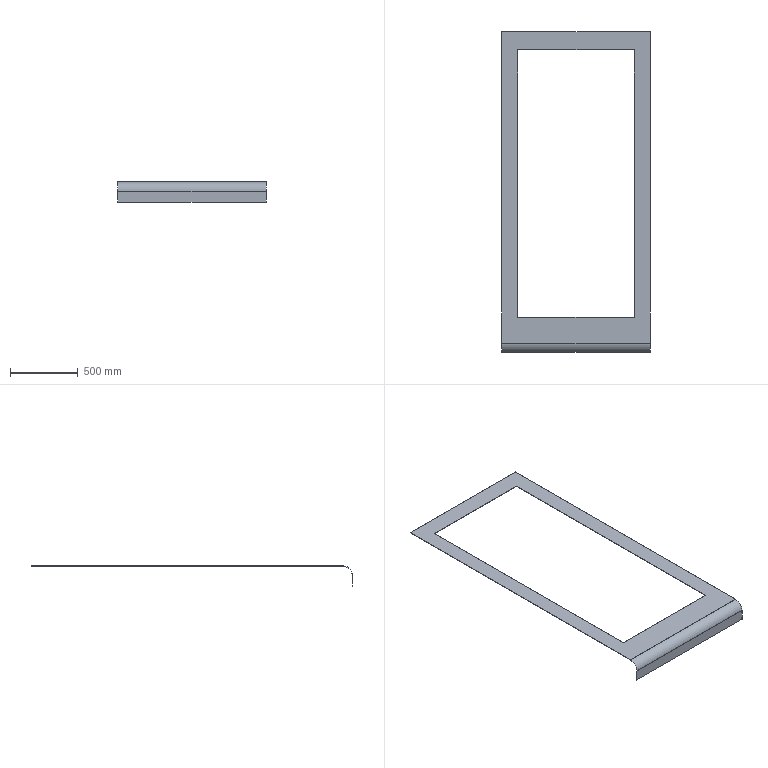Component | SolidWorks | A-SideAluminumCasingAssembly-1_A-SideAluminumCasing2-2 | 1 solid | 18 faces | box 1100 x 2375.5 x 149.5 mm | volume 3119177 mm3 | plane 16 | cylinder 2 | commonest cylinder face diameters 139 x1 133 x1
STEP:
#1=CARTESIAN_POINT('',(0.,0.,73.937));
#2=VERTEX_POINT('',#1);
#3=CARTESIAN_POINT('',(0.,0.,73.819));
#4=VERTEX_POINT('',#3);
#5=CARTESIAN_POINT('',(0.,0.,73.819));
#6=DIRECTION('',(0.,-0.,-1.));
#7=VECTOR('',#6,39.37);
#8=LINE('',#5,#7);
#9=EDGE_CURVE('',#2,#4,#8,.T.);
#10=ORIENTED_EDGE('',*,*,#9,.F.);
#11=CARTESIAN_POINT('',(-0.,90.787,73.937));
#12=VERTEX_POINT('',#11);
#13=CARTESIAN_POINT('',(0.,0.,73.937));
#14=DIRECTION('',(-0.,1.,-0.));
#15=VECTOR('',#14,39.37);
#16=LINE('',#13,#15);
#17=EDGE_CURVE('',#2,#12,#16,.T.);
#18=ORIENTED_EDGE('',*,*,#17,.T.);
#19=CARTESIAN_POINT('',(-0.,90.787,73.819));
#20=VERTEX_POINT('',#19);
#21=CARTESIAN_POINT('',(-0.,90.787,73.819));
#22=DIRECTION('',(0.,-0.,-1.));
#23=VECTOR('',#22,39.37);
#24=LINE('',#21,#23);
#25=EDGE_CURVE('',#12,#20,#24,.T.);
#26=ORIENTED_EDGE('',*,*,#25,.T.);
#27=CARTESIAN_POINT('',(0.,0.,73.819));
#28=DIRECTION('',(-0.,1.,-0.));
#29=VECTOR('',#28,39.37);
#30=LINE('',#27,#29);
#31=EDGE_CURVE('',#4,#20,#30,.T.);
#32=ORIENTED_EDGE('',*,*,#31,.F.);
#33=EDGE_LOOP('',(#10,#18,#26,#32));
#34=FACE_OUTER_BOUND('',#33,.T.);
#35=CARTESIAN_POINT('',(0.,0.,73.819));
#36=DIRECTION('',(1.,0.,0.));
#37=DIRECTION('',(-0.,1.,-0.));
#38=AXIS2_PLACEMENT_3D('',#35,#36,#37);
#39=PLANE('',#38);
#40=ADVANCED_FACE('',(#34),#39,.F.);
#41=ORIENTED_EDGE('',*,*,#25,.F.);
#42=CARTESIAN_POINT('',(43.307,90.787,73.937));
#43=VERTEX_POINT('',#42);
#44=CARTESIAN_POINT('',(43.307,90.787,73.937));
#45=DIRECTION('',(1.,0.,0.));
#46=VECTOR('',#45,39.37);
#47=LINE('',#44,#46);
#48=EDGE_CURVE('',#12,#43,#47,.T.);
#49=ORIENTED_EDGE('',*,*,#48,.T.);
#50=CARTESIAN_POINT('',(43.307,90.787,73.819));
#51=VERTEX_POINT('',#50);
#52=CARTESIAN_POINT('',(43.307,90.787,73.819));
#53=DIRECTION('',(0.,-0.,-1.));
#54=VECTOR('',#53,39.37);
#55=LINE('',#52,#54);
#56=EDGE_CURVE('',#43,#51,#55,.T.);
#57=ORIENTED_EDGE('',*,*,#56,.T.);
#58=CARTESIAN_POINT('',(43.307,90.787,73.819));
#59=DIRECTION('',(1.,0.,0.));
#60=VECTOR('',#59,39.37);
#61=LINE('',#58,#60);
#62=EDGE_CURVE('',#20,#51,#61,.T.);
#63=ORIENTED_EDGE('',*,*,#62,.F.);
#64=EDGE_LOOP('',(#41,#49,#57,#63));
#65=FACE_OUTER_BOUND('',#64,.T.);
#66=CARTESIAN_POINT('',(43.307,90.787,73.819));
#67=DIRECTION('',(0.,-1.,0.));
#68=DIRECTION('',(1.,0.,0.));
#69=AXIS2_PLACEMENT_3D('',#66,#67,#68);
#70=PLANE('',#69);
#71=ADVANCED_FACE('',(#65),#70,.F.);
#72=ORIENTED_EDGE('',*,*,#56,.F.);
#73=CARTESIAN_POINT('',(43.307,0.,73.937));
#74=VERTEX_POINT('',#73);
#75=CARTESIAN_POINT('',(43.307,0.,73.937));
#76=DIRECTION('',(0.,-1.,0.));
#77=VECTOR('',#76,39.37);
#78=LINE('',#75,#77);
#79=EDGE_CURVE('',#43,#74,#78,.T.);
#80=ORIENTED_EDGE('',*,*,#79,.T.);
#81=CARTESIAN_POINT('',(43.307,0.,73.819));
#82=VERTEX_POINT('',#81);
#83=CARTESIAN_POINT('',(43.307,0.,73.819));
#84=DIRECTION('',(0.,-0.,-1.));
#85=VECTOR('',#84,39.37);
#86=LINE('',#83,#85);
#87=EDGE_CURVE('',#74,#82,#86,.T.);
#88=ORIENTED_EDGE('',*,*,#87,.T.);
#89=CARTESIAN_POINT('',(43.307,0.,73.819));
#90=DIRECTION('',(0.,-1.,0.));
#91=VECTOR('',#90,39.37);
#92=LINE('',#89,#91);
#93=EDGE_CURVE('',#51,#82,#92,.T.);
#94=ORIENTED_EDGE('',*,*,#93,.F.);
#95=EDGE_LOOP('',(#72,#80,#88,#94));
#96=FACE_OUTER_BOUND('',#95,.T.);
#97=CARTESIAN_POINT('',(43.307,0.,73.819));
#98=DIRECTION('',(-1.,-0.,-0.));
#99=DIRECTION('',(0.,-1.,0.));
#100=AXIS2_PLACEMENT_3D('',#97,#98,#99);
#101=PLANE('',#100);
#102=ADVANCED_FACE('',(#96),#101,.F.);
#103=CARTESIAN_POINT('',(38.583,85.413,73.819));
#104=VERTEX_POINT('',#103);
#105=CARTESIAN_POINT('',(4.724,85.413,73.819));
#106=VERTEX_POINT('',#105);
#107=CARTESIAN_POINT('',(43.307,85.413,73.819));
#108=DIRECTION('',(-1.,-0.,-0.));
#109=VECTOR('',#108,39.37);
#110=LINE('',#107,#109);
#111=EDGE_CURVE('',#104,#106,#110,.T.);
#112=ORIENTED_EDGE('',*,*,#111,.T.);
#113=CARTESIAN_POINT('',(4.724,7.48,73.819));
#114=VERTEX_POINT('',#113);
#115=CARTESIAN_POINT('',(4.724,0.,73.819));
#116=DIRECTION('',(0.,-1.,0.));
#117=VECTOR('',#116,39.37);
#118=LINE('',#115,#117);
#119=EDGE_CURVE('',#106,#114,#118,.T.);
#120=ORIENTED_EDGE('',*,*,#119,.T.);
#121=CARTESIAN_POINT('',(38.583,7.48,73.819));
#122=VERTEX_POINT('',#121);
#123=CARTESIAN_POINT('',(43.307,7.48,73.819));
#124=DIRECTION('',(1.,0.,0.));
#125=VECTOR('',#124,39.37);
#126=LINE('',#123,#125);
#127=EDGE_CURVE('',#114,#122,#126,.T.);
#128=ORIENTED_EDGE('',*,*,#127,.T.);
#129=CARTESIAN_POINT('',(38.583,0.,73.819));
#130=DIRECTION('',(-0.,1.,-0.));
#131=VECTOR('',#130,39.37);
#132=LINE('',#129,#131);
#133=EDGE_CURVE('',#122,#104,#132,.T.);
#134=ORIENTED_EDGE('',*,*,#133,.T.);
#135=EDGE_LOOP('',(#112,#120,#128,#134));
#136=FACE_BOUND('',#135,.T.);
#137=ORIENTED_EDGE('',*,*,#93,.T.);
#138=CARTESIAN_POINT('',(43.307,0.,73.819));
#139=DIRECTION('',(-1.,-0.,-0.));
#140=VECTOR('',#139,39.37);
#141=LINE('',#138,#140);
#142=EDGE_CURVE('',#82,#4,#141,.T.);
#143=ORIENTED_EDGE('',*,*,#142,.T.);
#144=ORIENTED_EDGE('',*,*,#31,.T.);
#145=ORIENTED_EDGE('',*,*,#62,.T.);
#146=EDGE_LOOP('',(#137,#143,#144,#145));
#147=FACE_OUTER_BOUND('',#146,.T.);
#148=CARTESIAN_POINT('',(43.307,0.,73.819));
#149=DIRECTION('',(-0.,0.,1.));
#150=DIRECTION('',(1.,0.,0.));
#151=AXIS2_PLACEMENT_3D('',#148,#149,#150);
#152=PLANE('',#151);
#153=ADVANCED_FACE('',(#136,#147),#152,.F.);
#154=CARTESIAN_POINT('',(4.724,85.413,73.937));
#155=VERTEX_POINT('',#154);
#156=CARTESIAN_POINT('',(4.724,7.48,73.937));
#157=VERTEX_POINT('',#156);
#158=CARTESIAN_POINT('',(4.724,85.413,73.937));
#159=DIRECTION('',(0.,-1.,0.));
#160=VECTOR('',#159,39.37);
#161=LINE('',#158,#160);
#162=EDGE_CURVE('',#155,#157,#161,.T.);
#163=ORIENTED_EDGE('',*,*,#162,.F.);
#164=CARTESIAN_POINT('',(38.583,85.413,73.937));
#165=VERTEX_POINT('',#164);
#166=CARTESIAN_POINT('',(4.724,85.413,73.937));
#167=DIRECTION('',(-1.,-0.,-0.));
#168=VECTOR('',#167,39.37);
#169=LINE('',#166,#168);
#170=EDGE_CURVE('',#165,#155,#169,.T.);
#171=ORIENTED_EDGE('',*,*,#170,.F.);
#172=CARTESIAN_POINT('',(38.583,7.48,73.937));
#173=VERTEX_POINT('',#172);
#174=CARTESIAN_POINT('',(38.583,85.413,73.937));
#175=DIRECTION('',(-0.,1.,-0.));
#176=VECTOR('',#175,39.37);
#177=LINE('',#174,#176);
#178=EDGE_CURVE('',#173,#165,#177,.T.);
#179=ORIENTED_EDGE('',*,*,#178,.F.);
#180=CARTESIAN_POINT('',(4.724,7.48,73.937));
#181=DIRECTION('',(1.,0.,0.));
#182=VECTOR('',#181,39.37);
#183=LINE('',#180,#182);
#184=EDGE_CURVE('',#157,#173,#183,.T.);
#185=ORIENTED_EDGE('',*,*,#184,.F.);
#186=EDGE_LOOP('',(#163,#171,#179,#185));
#187=FACE_BOUND('',#186,.T.);
#188=ORIENTED_EDGE('',*,*,#79,.F.);
#189=ORIENTED_EDGE('',*,*,#48,.F.);
#190=ORIENTED_EDGE('',*,*,#17,.F.);
#191=CARTESIAN_POINT('',(43.307,0.,73.937));
#192=DIRECTION('',(-1.,-0.,-0.));
#193=VECTOR('',#192,39.37);
#194=LINE('',#191,#193);
#195=EDGE_CURVE('',#74,#2,#194,.T.);
#196=ORIENTED_EDGE('',*,*,#195,.F.);
#197=EDGE_LOOP('',(#188,#189,#190,#196));
#198=FACE_OUTER_BOUND('',#197,.T.);
#199=CARTESIAN_POINT('',(43.307,0.,73.937));
#200=DIRECTION('',(-0.,0.,1.));
#201=DIRECTION('',(1.,0.,0.));
#202=AXIS2_PLACEMENT_3D('',#199,#200,#201);
#203=PLANE('',#202);
#204=ADVANCED_FACE('',(#187,#198),#203,.T.);
#205=CARTESIAN_POINT('',(43.307,-2.618,71.201));
#206=VERTEX_POINT('',#205);
#207=CARTESIAN_POINT('',(43.307,-2.736,71.201));
#208=VERTEX_POINT('',#207);
#209=CARTESIAN_POINT('',(43.307,-2.736,71.201));
#210=DIRECTION('',(0.,-1.,0.));
#211=VECTOR('',#210,39.37);
#212=LINE('',#209,#211);
#213=EDGE_CURVE('',#206,#208,#212,.T.);
#214=ORIENTED_EDGE('',*,*,#213,.F.);
#215=CARTESIAN_POINT('',(43.307,0.,71.201));
#216=DIRECTION('',(1.,0.,0.));
#217=DIRECTION('',(0.,0.,1.));
#218=AXIS2_PLACEMENT_3D('',#215,#216,#217);
#219=CIRCLE('',#218,2.618);
#220=EDGE_CURVE('',#82,#206,#219,.T.);
#221=ORIENTED_EDGE('',*,*,#220,.F.);
#222=ORIENTED_EDGE('',*,*,#87,.F.);
#223=CARTESIAN_POINT('',(43.307,0.,71.201));
#224=DIRECTION('',(1.,0.,0.));
#225=DIRECTION('',(0.,0.,1.));
#226=AXIS2_PLACEMENT_3D('',#223,#224,#225);
#227=CIRCLE('',#226,2.736);
#228=EDGE_CURVE('',#74,#208,#227,.T.);
#229=ORIENTED_EDGE('',*,*,#228,.T.);
#230=EDGE_LOOP('',(#214,#221,#222,#229));
#231=FACE_OUTER_BOUND('',#230,.T.);
#232=CARTESIAN_POINT('',(43.307,0.,71.201));
#233=DIRECTION('',(1.,0.,0.));
#234=DIRECTION('',(0.,-0.,-1.));
#235=AXIS2_PLACEMENT_3D('',#232,#233,#234);
#236=PLANE('',#235);
#237=ADVANCED_FACE('',(#231),#236,.T.);
#238=CARTESIAN_POINT('',(0.,-2.618,71.201));
#239=VERTEX_POINT('',#238);
#240=CARTESIAN_POINT('',(0.,0.,71.201));
#241=DIRECTION('',(-1.,-0.,-0.));
#242=DIRECTION('',(-0.,0.,1.));
#243=AXIS2_PLACEMENT_3D('',#240,#241,#242);
#244=CIRCLE('',#243,2.618);
#245=EDGE_CURVE('',#239,#4,#244,.T.);
#246=ORIENTED_EDGE('',*,*,#245,.F.);
#247=CARTESIAN_POINT('',(0.,-2.736,71.201));
#248=VERTEX_POINT('',#247);
#249=CARTESIAN_POINT('',(0.,-2.618,71.201));
#250=DIRECTION('',(0.,-1.,0.));
#251=VECTOR('',#250,39.37);
#252=LINE('',#249,#251);
#253=EDGE_CURVE('',#239,#248,#252,.T.);
#254=ORIENTED_EDGE('',*,*,#253,.T.);
#255=CARTESIAN_POINT('',(0.,0.,71.201));
#256=DIRECTION('',(-1.,-0.,-0.));
#257=DIRECTION('',(-0.,0.,1.));
#258=AXIS2_PLACEMENT_3D('',#255,#256,#257);
#259=CIRCLE('',#258,2.736);
#260=EDGE_CURVE('',#248,#2,#259,.T.);
#261=ORIENTED_EDGE('',*,*,#260,.T.);
#262=ORIENTED_EDGE('',*,*,#9,.T.);
#263=EDGE_LOOP('',(#246,#254,#261,#262));
#264=FACE_OUTER_BOUND('',#263,.T.);
#265=CARTESIAN_POINT('',(0.,0.,71.201));
#266=DIRECTION('',(1.,0.,0.));
#267=DIRECTION('',(0.,-0.,-1.));
#268=AXIS2_PLACEMENT_3D('',#265,#266,#267);
#269=PLANE('',#268);
#270=ADVANCED_FACE('',(#264),#269,.F.);
#271=ORIENTED_EDGE('',*,*,#195,.T.);
#272=ORIENTED_EDGE('',*,*,#260,.F.);
#273=CARTESIAN_POINT('',(43.307,-2.736,71.201));
#274=DIRECTION('',(-1.,-0.,-0.));
#275=VECTOR('',#274,39.37);
#276=LINE('',#273,#275);
#277=EDGE_CURVE('',#208,#248,#276,.T.);
#278=ORIENTED_EDGE('',*,*,#277,.F.);
#279=ORIENTED_EDGE('',*,*,#228,.F.);
#280=EDGE_LOOP('',(#271,#272,#278,#279));
#281=FACE_OUTER_BOUND('',#280,.T.);
#282=CARTESIAN_POINT('',(0.,0.,71.201));
#283=DIRECTION('',(-1.,-0.,-0.));
#284=DIRECTION('',(0.,-1.,0.));
#285=AXIS2_PLACEMENT_3D('',#282,#283,#284);
#286=CYLINDRICAL_SURFACE('',#285,2.736);
#287=ADVANCED_FACE('',(#281),#286,.T.);
#288=ORIENTED_EDGE('',*,*,#142,.F.);
#289=ORIENTED_EDGE('',*,*,#220,.T.);
#290=CARTESIAN_POINT('',(43.307,-2.618,71.201));
#291=DIRECTION('',(-1.,-0.,-0.));
#292=VECTOR('',#291,39.37);
#293=LINE('',#290,#292);
#294=EDGE_CURVE('',#206,#239,#293,.T.);
#295=ORIENTED_EDGE('',*,*,#294,.T.);
#296=ORIENTED_EDGE('',*,*,#245,.T.);
#297=EDGE_LOOP('',(#288,#289,#295,#296));
#298=FACE_OUTER_BOUND('',#297,.T.);
#299=CARTESIAN_POINT('',(0.,0.,71.201));
#300=DIRECTION('',(-1.,-0.,-0.));
#301=DIRECTION('',(0.,-1.,0.));
#302=AXIS2_PLACEMENT_3D('',#299,#300,#301);
#303=CYLINDRICAL_SURFACE('',#302,2.618);
#304=ADVANCED_FACE('',(#298),#303,.F.);
#305=CARTESIAN_POINT('',(0.,-2.736,68.051));
#306=VERTEX_POINT('',#305);
#307=CARTESIAN_POINT('',(0.,-2.736,73.819));
#308=DIRECTION('',(-0.,0.,1.));
#309=VECTOR('',#308,39.37);
#310=LINE('',#307,#309);
#311=EDGE_CURVE('',#306,#248,#310,.T.);
#312=ORIENTED_EDGE('',*,*,#311,.T.);
#313=ORIENTED_EDGE('',*,*,#253,.F.);
#314=CARTESIAN_POINT('',(0.,-2.618,68.051));
#315=VERTEX_POINT('',#314);
#316=CARTESIAN_POINT('',(0.,-2.618,73.819));
#317=DIRECTION('',(-0.,0.,1.));
#318=VECTOR('',#317,39.37);
#319=LINE('',#316,#318);
#320=EDGE_CURVE('',#315,#239,#319,.T.);
#321=ORIENTED_EDGE('',*,*,#320,.F.);
#322=CARTESIAN_POINT('',(0.,-2.736,68.051));
#323=DIRECTION('',(-0.,1.,-0.));
#324=VECTOR('',#323,39.37);
#325=LINE('',#322,#324);
#326=EDGE_CURVE('',#306,#315,#325,.T.);
#327=ORIENTED_EDGE('',*,*,#326,.F.);
#328=EDGE_LOOP('',(#312,#313,#321,#327));
#329=FACE_OUTER_BOUND('',#328,.T.);
#330=CARTESIAN_POINT('',(0.,-2.736,73.819));
#331=DIRECTION('',(-1.,-0.,-0.));
#332=DIRECTION('',(-0.,0.,1.));
#333=AXIS2_PLACEMENT_3D('',#330,#331,#332);
#334=PLANE('',#333);
#335=ADVANCED_FACE('',(#329),#334,.T.);
#336=CARTESIAN_POINT('',(43.307,-2.618,68.051));
#337=VERTEX_POINT('',#336);
#338=CARTESIAN_POINT('',(43.307,-2.618,73.819));
#339=DIRECTION('',(0.,-0.,-1.));
#340=VECTOR('',#339,39.37);
#341=LINE('',#338,#340);
#342=EDGE_CURVE('',#206,#337,#341,.T.);
#343=ORIENTED_EDGE('',*,*,#342,.F.);
#344=ORIENTED_EDGE('',*,*,#213,.T.);
#345=CARTESIAN_POINT('',(43.307,-2.736,68.051));
#346=VERTEX_POINT('',#345);
#347=CARTESIAN_POINT('',(43.307,-2.736,68.051));
#348=DIRECTION('',(0.,-0.,-1.));
#349=VECTOR('',#348,39.37);
#350=LINE('',#347,#349);
#351=EDGE_CURVE('',#208,#346,#350,.T.);
#352=ORIENTED_EDGE('',*,*,#351,.T.);
#353=CARTESIAN_POINT('',(43.307,-2.736,68.051));
#354=DIRECTION('',(-0.,1.,-0.));
#355=VECTOR('',#354,39.37);
#356=LINE('',#353,#355);
#357=EDGE_CURVE('',#346,#337,#356,.T.);
#358=ORIENTED_EDGE('',*,*,#357,.T.);
#359=EDGE_LOOP('',(#343,#344,#352,#358));
#360=FACE_OUTER_BOUND('',#359,.T.);
#361=CARTESIAN_POINT('',(43.307,-2.736,68.051));
#362=DIRECTION('',(1.,0.,0.));
#363=DIRECTION('',(0.,-0.,-1.));
#364=AXIS2_PLACEMENT_3D('',#361,#362,#363);
#365=PLANE('',#364);
#366=ADVANCED_FACE('',(#360),#365,.T.);
#367=ORIENTED_EDGE('',*,*,#351,.F.);
#368=ORIENTED_EDGE('',*,*,#277,.T.);
#369=ORIENTED_EDGE('',*,*,#311,.F.);
#370=CARTESIAN_POINT('',(0.,-2.736,68.051));
#371=DIRECTION('',(-1.,-0.,-0.));
#372=VECTOR('',#371,39.37);
#373=LINE('',#370,#372);
#374=EDGE_CURVE('',#346,#306,#373,.T.);
#375=ORIENTED_EDGE('',*,*,#374,.F.);
#376=EDGE_LOOP('',(#367,#368,#369,#375));
#377=FACE_OUTER_BOUND('',#376,.T.);
#378=CARTESIAN_POINT('',(43.307,-2.736,73.819));
#379=DIRECTION('',(0.,-1.,0.));
#380=DIRECTION('',(-0.,0.,1.));
#381=AXIS2_PLACEMENT_3D('',#378,#379,#380);
#382=PLANE('',#381);
#383=ADVANCED_FACE('',(#377),#382,.T.);
#384=ORIENTED_EDGE('',*,*,#294,.F.);
#385=ORIENTED_EDGE('',*,*,#342,.T.);
#386=CARTESIAN_POINT('',(43.307,-2.618,68.051));
#387=DIRECTION('',(-1.,-0.,-0.));
#388=VECTOR('',#387,39.37);
#389=LINE('',#386,#388);
#390=EDGE_CURVE('',#337,#315,#389,.T.);
#391=ORIENTED_EDGE('',*,*,#390,.T.);
#392=ORIENTED_EDGE('',*,*,#320,.T.);
#393=EDGE_LOOP('',(#384,#385,#391,#392));
#394=FACE_OUTER_BOUND('',#393,.T.);
#395=CARTESIAN_POINT('',(43.307,-2.618,73.819));
#396=DIRECTION('',(0.,-1.,0.));
#397=DIRECTION('',(-0.,0.,1.));
#398=AXIS2_PLACEMENT_3D('',#395,#396,#397);
#399=PLANE('',#398);
#400=ADVANCED_FACE('',(#394),#399,.F.);
#401=ORIENTED_EDGE('',*,*,#390,.F.);
#402=ORIENTED_EDGE('',*,*,#357,.F.);
#403=ORIENTED_EDGE('',*,*,#374,.T.);
#404=ORIENTED_EDGE('',*,*,#326,.T.);
#405=EDGE_LOOP('',(#401,#402,#403,#404));
#406=FACE_OUTER_BOUND('',#405,.T.);
#407=CARTESIAN_POINT('',(0.,-2.736,68.051));
#408=DIRECTION('',(0.,-0.,-1.));
#409=DIRECTION('',(0.,-1.,0.));
#410=AXIS2_PLACEMENT_3D('',#407,#408,#409);
#411=PLANE('',#410);
#412=ADVANCED_FACE('',(#406),#411,.T.);
#413=CARTESIAN_POINT('',(4.724,85.413,68.051));
#414=DIRECTION('',(-0.,0.,1.));
#415=VECTOR('',#414,39.37);
#416=LINE('',#413,#415);
#417=EDGE_CURVE('',#106,#155,#416,.T.);
#418=ORIENTED_EDGE('',*,*,#417,.T.);
#419=ORIENTED_EDGE('',*,*,#162,.T.);
#420=CARTESIAN_POINT('',(4.724,7.48,68.051));
#421=DIRECTION('',(-0.,0.,1.));
#422=VECTOR('',#421,39.37);
#423=LINE('',#420,#422);
#424=EDGE_CURVE('',#114,#157,#423,.T.);
#425=ORIENTED_EDGE('',*,*,#424,.F.);
#426=ORIENTED_EDGE('',*,*,#119,.F.);
#427=EDGE_LOOP('',(#418,#419,#425,#426));
#428=FACE_OUTER_BOUND('',#427,.T.);
#429=CARTESIAN_POINT('',(4.724,85.413,68.051));
#430=DIRECTION('',(-1.,-0.,-0.));
#431=DIRECTION('',(-0.,1.,-0.));
#432=AXIS2_PLACEMENT_3D('',#429,#430,#431);
#433=PLANE('',#432);
#434=ADVANCED_FACE('',(#428),#433,.F.);
#435=CARTESIAN_POINT('',(38.583,85.413,68.051));
#436=DIRECTION('',(-0.,0.,1.));
#437=VECTOR('',#436,39.37);
#438=LINE('',#435,#437);
#439=EDGE_CURVE('',#104,#165,#438,.T.);
#440=ORIENTED_EDGE('',*,*,#439,.T.);
#441=ORIENTED_EDGE('',*,*,#170,.T.);
#442=ORIENTED_EDGE('',*,*,#417,.F.);
#443=ORIENTED_EDGE('',*,*,#111,.F.);
#444=EDGE_LOOP('',(#440,#441,#442,#443));
#445=FACE_OUTER_BOUND('',#444,.T.);
#446=CARTESIAN_POINT('',(4.724,85.413,68.051));
#447=DIRECTION('',(-0.,1.,-0.));
#448=DIRECTION('',(0.,-0.,-1.));
#449=AXIS2_PLACEMENT_3D('',#446,#447,#448);
#450=PLANE('',#449);
#451=ADVANCED_FACE('',(#445),#450,.F.);
#452=CARTESIAN_POINT('',(38.583,7.48,68.051));
#453=DIRECTION('',(-0.,0.,1.));
#454=VECTOR('',#453,39.37);
#455=LINE('',#452,#454);
#456=EDGE_CURVE('',#122,#173,#455,.T.);
#457=ORIENTED_EDGE('',*,*,#456,.T.);
#458=ORIENTED_EDGE('',*,*,#178,.T.);
#459=ORIENTED_EDGE('',*,*,#439,.F.);
#460=ORIENTED_EDGE('',*,*,#133,.F.);
#461=EDGE_LOOP('',(#457,#458,#459,#460));
#462=FACE_OUTER_BOUND('',#461,.T.);
#463=CARTESIAN_POINT('',(38.583,85.413,68.051));
#464=DIRECTION('',(1.,0.,0.));
#465=DIRECTION('',(0.,-1.,0.));
#466=AXIS2_PLACEMENT_3D('',#463,#464,#465);
#467=PLANE('',#466);
#468=ADVANCED_FACE('',(#462),#467,.F.);
#469=ORIENTED_EDGE('',*,*,#424,.T.);
#470=ORIENTED_EDGE('',*,*,#184,.T.);
#471=ORIENTED_EDGE('',*,*,#456,.F.);
#472=ORIENTED_EDGE('',*,*,#127,.F.);
#473=EDGE_LOOP('',(#469,#470,#471,#472));
#474=FACE_OUTER_BOUND('',#473,.T.);
#475=CARTESIAN_POINT('',(4.724,7.48,68.051));
#476=DIRECTION('',(0.,-1.,0.));
#477=DIRECTION('',(-0.,0.,1.));
#478=AXIS2_PLACEMENT_3D('',#475,#476,#477);
#479=PLANE('',#478);
#480=ADVANCED_FACE('',(#474),#479,.F.);
#481=CLOSED_SHELL('',(#40,#71,#102,#153,#204,#237,#270,#287,#304,#335,#366,#383,#400,#412,#434,#451,#468,#480));
#482=MANIFOLD_SOLID_BREP('',#481);
#483=CARTESIAN_POINT('',(0.,0.,0.));
#484=DIRECTION('',(0.,0.,1.));
#485=DIRECTION('',(1.,0.,0.));
#486=AXIS2_PLACEMENT_3D('',#483,#484,#485);
#487=(LENGTH_UNIT()NAMED_UNIT(*)SI_UNIT($,.METRE.));
#488=LENGTH_MEASURE_WITH_UNIT(LENGTH_MEASURE(0.0254),#487);
#489=DIMENSIONAL_EXPONENTS(1.,0.,0.,0.,0.,0.,0.);
#490=(CONVERSION_BASED_UNIT('',#488)LENGTH_UNIT()NAMED_UNIT(#489));
#491=UNCERTAINTY_MEASURE_WITH_UNIT(LENGTH_MEASURE(0.00001),#490,'','');
#492=(NAMED_UNIT(*)PLANE_ANGLE_UNIT()SI_UNIT($,.RADIAN.));
#493=(NAMED_UNIT(*)SI_UNIT($,.STERADIAN.)SOLID_ANGLE_UNIT());
#494=(GEOMETRIC_REPRESENTATION_CONTEXT(3)GLOBAL_UNCERTAINTY_ASSIGNED_CONTEXT((#491))GLOBAL_UNIT_ASSIGNED_CONTEXT((#490,#492,#493))REPRESENTATION_CONTEXT('',''));
#495=ADVANCED_BREP_SHAPE_REPRESENTATION('',(#482,#486),#494);
#496=COLOUR_RGB('',0.7922,0.8196,0.9333);
#497=FILL_AREA_STYLE_COLOUR('',#496);
#498=FILL_AREA_STYLE('',(#497));
#499=SURFACE_STYLE_FILL_AREA(#498);
#500=SURFACE_SIDE_STYLE('',(#499));
#501=SURFACE_STYLE_USAGE(.BOTH.,#500);
#502=PRESENTATION_STYLE_ASSIGNMENT((#501));
#503=STYLED_ITEM('',(#502),#482);
#504=PRESENTATION_LAYER_ASSIGNMENT('','',(#503));
#505=(LENGTH_UNIT()NAMED_UNIT(*)SI_UNIT($,.METRE.));
#506=LENGTH_MEASURE_WITH_UNIT(LENGTH_MEASURE(0.0254),#505);
#507=DIMENSIONAL_EXPONENTS(1.,0.,0.,0.,0.,0.,0.);
#508=(CONVERSION_BASED_UNIT('',#506)LENGTH_UNIT()NAMED_UNIT(#507));
#509=UNCERTAINTY_MEASURE_WITH_UNIT(LENGTH_MEASURE(0.00001),#508,'','');
#510=(NAMED_UNIT(*)PLANE_ANGLE_UNIT()SI_UNIT($,.RADIAN.));
#511=(NAMED_UNIT(*)SI_UNIT($,.STERADIAN.)SOLID_ANGLE_UNIT());
#512=(GEOMETRIC_REPRESENTATION_CONTEXT(3)GLOBAL_UNCERTAINTY_ASSIGNED_CONTEXT((#509))GLOBAL_UNIT_ASSIGNED_CONTEXT((#508,#510,#511))REPRESENTATION_CONTEXT('',''));
#513=MECHANICAL_DESIGN_GEOMETRIC_PRESENTATION_REPRESENTATION('',(#503),#512);